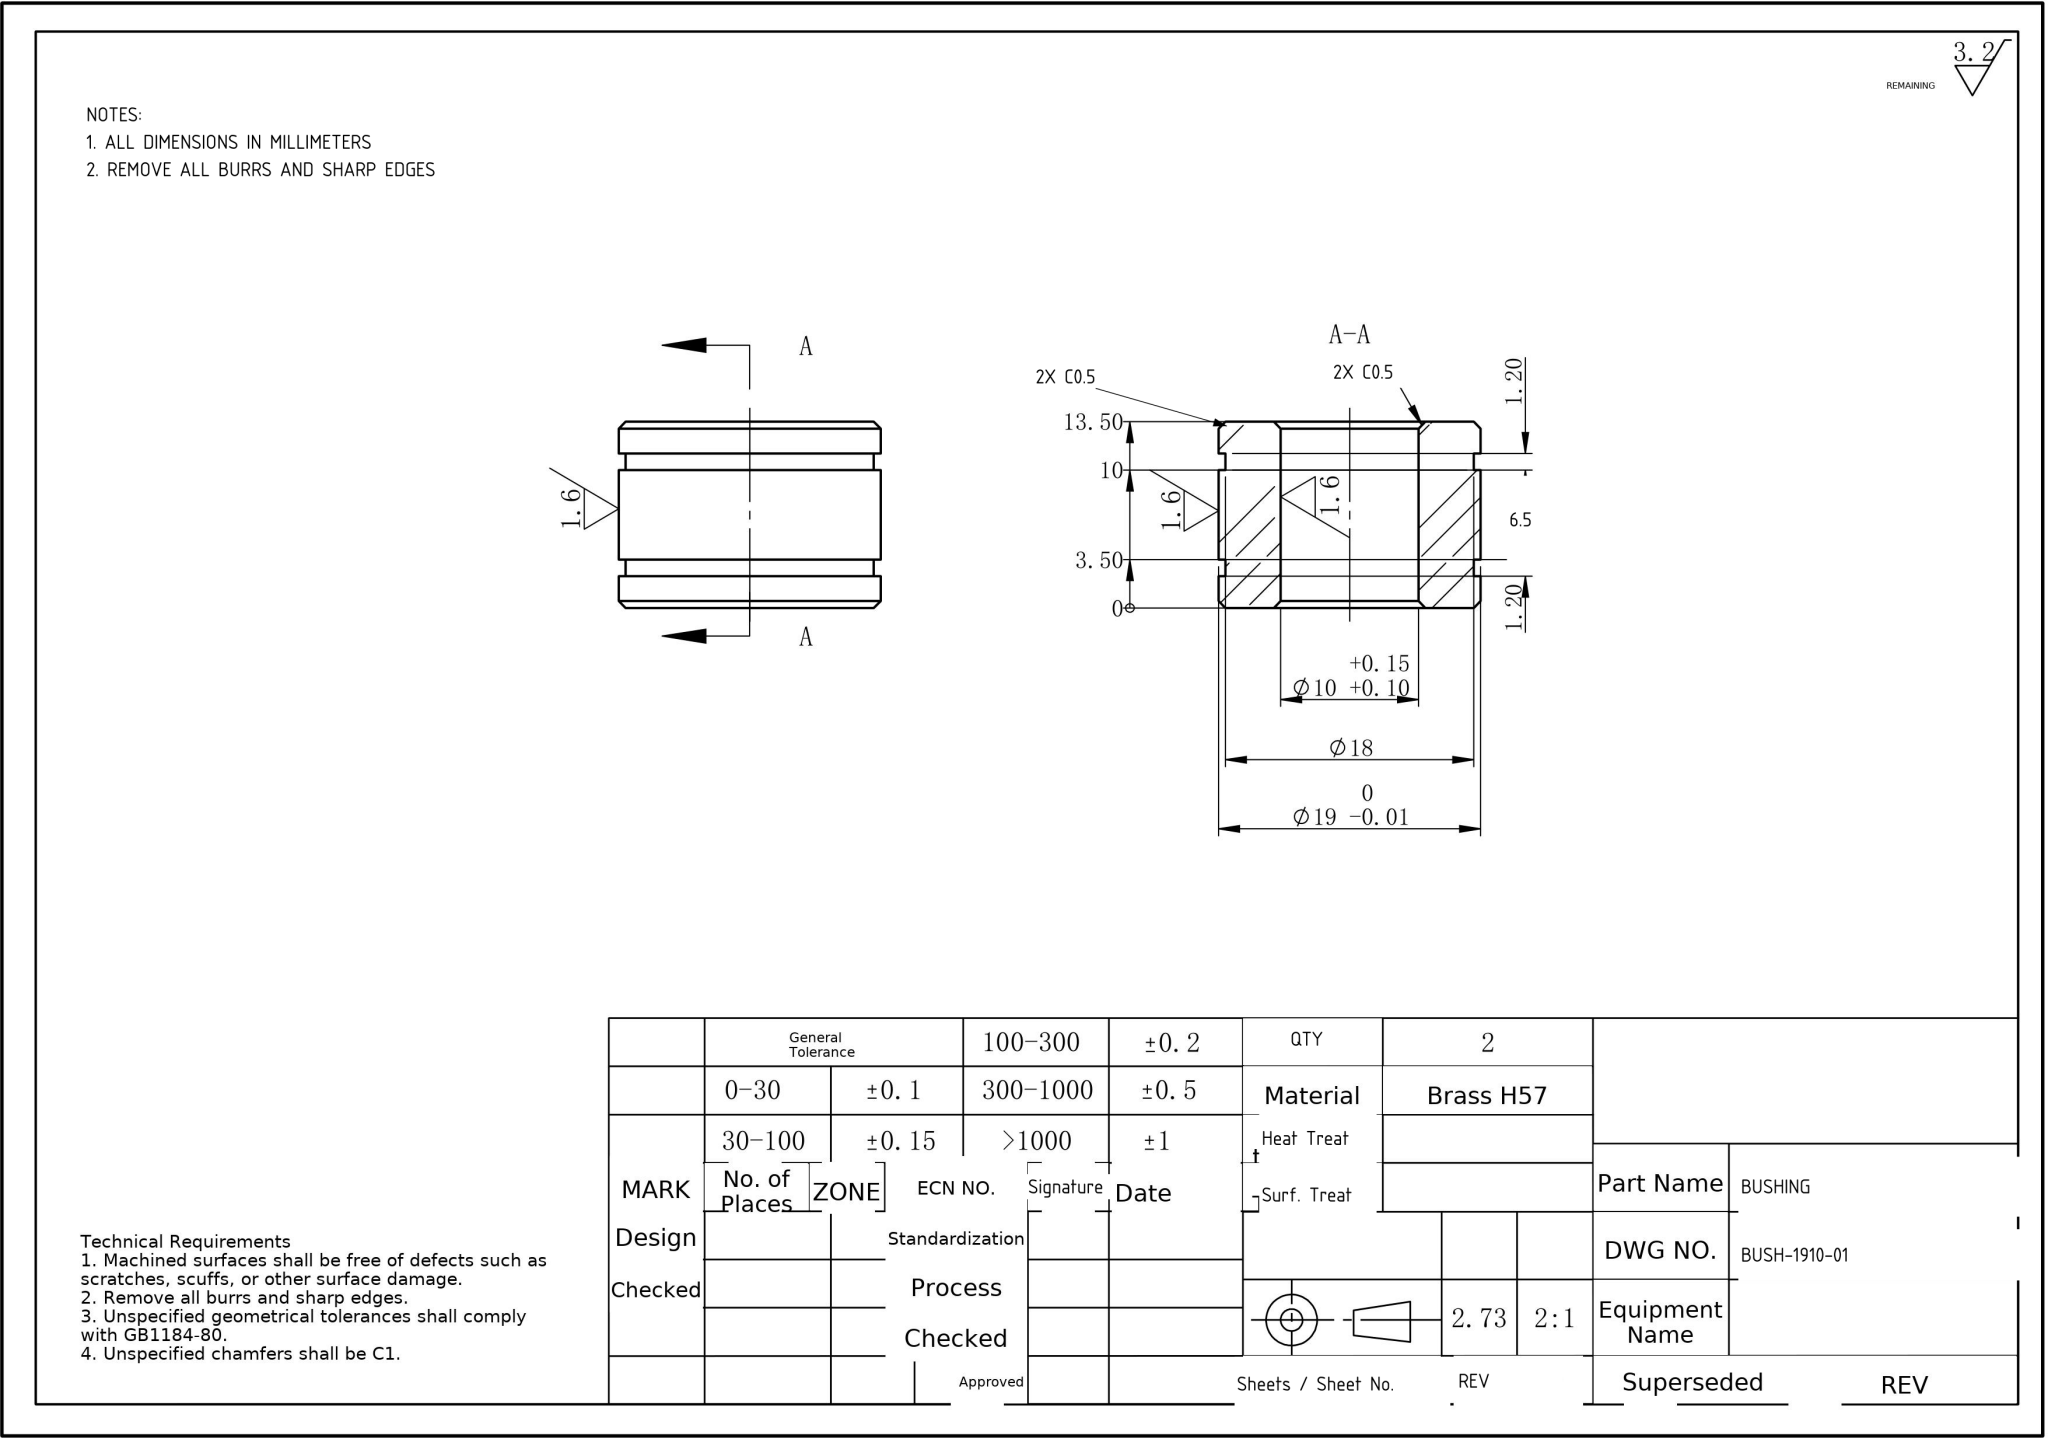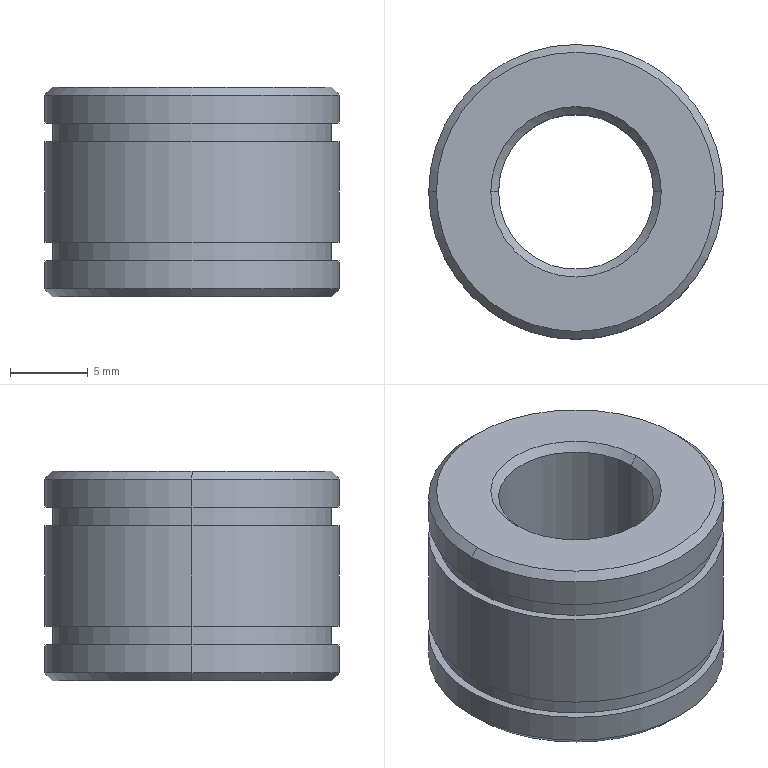Part | NX | mm | 1 solid | 26 faces | box 19 x 19 x 13.5 mm | volume 2675 mm3 | cylinder 12 | cone 8 | plane 6 | commonest cylinder face diameters 19 x6 18 x4 10 x2
STEP:
#1=COLOUR_RGB('',0.7922,0.8196,0.9333);
#2=FILL_AREA_STYLE_COLOUR('',#1);
#3=FILL_AREA_STYLE('',(#2));
#4=SURFACE_STYLE_FILL_AREA(#3);
#5=SURFACE_SIDE_STYLE('',(#4));
#6=SURFACE_STYLE_USAGE(.BOTH.,#5);
#7=PRESENTATION_STYLE_ASSIGNMENT((#6));
#8=CARTESIAN_POINT('',(-9.,0.,14.2));
#9=VERTEX_POINT('',#8);
#10=CARTESIAN_POINT('',(9.,0.,14.2));
#11=VERTEX_POINT('',#10);
#12=CARTESIAN_POINT('',(0.,0.,14.2));
#13=DIRECTION('',(0.,0.,-1.));
#14=DIRECTION('',(-1.,0.,0.));
#15=AXIS2_PLACEMENT_3D('',#12,#13,#14);
#16=CIRCLE('',#15,9.);
#17=EDGE_CURVE('',#9,#11,#16,.T.);
#18=ORIENTED_EDGE('',*,*,#17,.F.);
#19=CARTESIAN_POINT('',(-9.5,0.,14.7));
#20=VERTEX_POINT('',#19);
#21=CARTESIAN_POINT('',(-9.5,0.,14.7));
#22=DIRECTION('',(-0.7071,0.,0.7071));
#23=VECTOR('',#22,1000.);
#24=LINE('',#21,#23);
#25=EDGE_CURVE('',#9,#20,#24,.T.);
#26=ORIENTED_EDGE('',*,*,#25,.T.);
#27=CARTESIAN_POINT('',(9.5,0.,14.7));
#28=VERTEX_POINT('',#27);
#29=CARTESIAN_POINT('',(0.,0.,14.7));
#30=DIRECTION('',(0.,0.,1.));
#31=DIRECTION('',(-1.,0.,0.));
#32=AXIS2_PLACEMENT_3D('',#29,#30,#31);
#33=CIRCLE('',#32,9.5);
#34=EDGE_CURVE('',#28,#20,#33,.T.);
#35=ORIENTED_EDGE('',*,*,#34,.F.);
#36=CARTESIAN_POINT('',(9.5,0.,14.7));
#37=DIRECTION('',(0.7071,0.,0.7071));
#38=VECTOR('',#37,1000.);
#39=LINE('',#36,#38);
#40=EDGE_CURVE('',#11,#28,#39,.T.);
#41=ORIENTED_EDGE('',*,*,#40,.F.);
#42=EDGE_LOOP('',(#18,#26,#35,#41));
#43=FACE_OUTER_BOUND('',#42,.T.);
#44=CARTESIAN_POINT('',(0.,0.,14.7));
#45=DIRECTION('',(0.,0.,1.));
#46=DIRECTION('',(1.,0.,0.));
#47=AXIS2_PLACEMENT_3D('',#44,#45,#46);
#48=CONICAL_SURFACE('',#47,9.5,0.7854);
#49=ADVANCED_FACE('',(#43),#48,.T.);
#50=CARTESIAN_POINT('',(5.,0.,14.7));
#51=VERTEX_POINT('',#50);
#52=CARTESIAN_POINT('',(-5.,0.,14.7));
#53=VERTEX_POINT('',#52);
#54=CARTESIAN_POINT('',(0.,0.,14.7));
#55=DIRECTION('',(0.,0.,-1.));
#56=DIRECTION('',(-1.,0.,0.));
#57=AXIS2_PLACEMENT_3D('',#54,#55,#56);
#58=CIRCLE('',#57,5.);
#59=EDGE_CURVE('',#51,#53,#58,.T.);
#60=ORIENTED_EDGE('',*,*,#59,.F.);
#61=CARTESIAN_POINT('',(5.5,0.,14.2));
#62=VERTEX_POINT('',#61);
#63=CARTESIAN_POINT('',(5.5,0.,14.2));
#64=DIRECTION('',(0.7071,0.,-0.7071));
#65=VECTOR('',#64,1000.);
#66=LINE('',#63,#65);
#67=EDGE_CURVE('',#51,#62,#66,.T.);
#68=ORIENTED_EDGE('',*,*,#67,.T.);
#69=CARTESIAN_POINT('',(-5.5,0.,14.2));
#70=VERTEX_POINT('',#69);
#71=CARTESIAN_POINT('',(0.,0.,14.2));
#72=DIRECTION('',(0.,0.,1.));
#73=DIRECTION('',(-1.,0.,0.));
#74=AXIS2_PLACEMENT_3D('',#71,#72,#73);
#75=CIRCLE('',#74,5.5);
#76=EDGE_CURVE('',#70,#62,#75,.T.);
#77=ORIENTED_EDGE('',*,*,#76,.F.);
#78=CARTESIAN_POINT('',(-5.5,0.,14.2));
#79=DIRECTION('',(-0.7071,0.,-0.7071));
#80=VECTOR('',#79,1000.);
#81=LINE('',#78,#80);
#82=EDGE_CURVE('',#53,#70,#81,.T.);
#83=ORIENTED_EDGE('',*,*,#82,.F.);
#84=EDGE_LOOP('',(#60,#68,#77,#83));
#85=FACE_OUTER_BOUND('',#84,.T.);
#86=CARTESIAN_POINT('',(0.,0.,14.2));
#87=DIRECTION('',(0.,0.,-1.));
#88=DIRECTION('',(-1.,0.,0.));
#89=AXIS2_PLACEMENT_3D('',#86,#87,#88);
#90=CONICAL_SURFACE('',#89,5.5,0.7854);
#91=ADVANCED_FACE('',(#85),#90,.F.);
#92=CARTESIAN_POINT('',(9.,0.,27.7));
#93=VERTEX_POINT('',#92);
#94=CARTESIAN_POINT('',(-9.,0.,27.7));
#95=VERTEX_POINT('',#94);
#96=CARTESIAN_POINT('',(0.,0.,27.7));
#97=DIRECTION('',(0.,0.,1.));
#98=DIRECTION('',(1.,0.,0.));
#99=AXIS2_PLACEMENT_3D('',#96,#97,#98);
#100=CIRCLE('',#99,9.);
#101=EDGE_CURVE('',#93,#95,#100,.T.);
#102=ORIENTED_EDGE('',*,*,#101,.F.);
#103=CARTESIAN_POINT('',(9.5,0.,27.2));
#104=VERTEX_POINT('',#103);
#105=CARTESIAN_POINT('',(9.5,0.,27.2));
#106=DIRECTION('',(0.7071,0.,-0.7071));
#107=VECTOR('',#106,1000.);
#108=LINE('',#105,#107);
#109=EDGE_CURVE('',#93,#104,#108,.T.);
#110=ORIENTED_EDGE('',*,*,#109,.T.);
#111=CARTESIAN_POINT('',(-9.5,0.,27.2));
#112=VERTEX_POINT('',#111);
#113=CARTESIAN_POINT('',(0.,0.,27.2));
#114=DIRECTION('',(0.,0.,-1.));
#115=DIRECTION('',(1.,0.,0.));
#116=AXIS2_PLACEMENT_3D('',#113,#114,#115);
#117=CIRCLE('',#116,9.5);
#118=EDGE_CURVE('',#112,#104,#117,.T.);
#119=ORIENTED_EDGE('',*,*,#118,.F.);
#120=CARTESIAN_POINT('',(-9.5,0.,27.2));
#121=DIRECTION('',(-0.7071,0.,-0.7071));
#122=VECTOR('',#121,1000.);
#123=LINE('',#120,#122);
#124=EDGE_CURVE('',#95,#112,#123,.T.);
#125=ORIENTED_EDGE('',*,*,#124,.F.);
#126=EDGE_LOOP('',(#102,#110,#119,#125));
#127=FACE_OUTER_BOUND('',#126,.T.);
#128=CARTESIAN_POINT('',(0.,0.,27.2));
#129=DIRECTION('',(0.,0.,-1.));
#130=DIRECTION('',(-1.,0.,0.));
#131=AXIS2_PLACEMENT_3D('',#128,#129,#130);
#132=CONICAL_SURFACE('',#131,9.5,0.7854);
#133=ADVANCED_FACE('',(#127),#132,.T.);
#134=CARTESIAN_POINT('',(-5.,0.,27.2));
#135=VERTEX_POINT('',#134);
#136=CARTESIAN_POINT('',(5.,0.,27.2));
#137=VERTEX_POINT('',#136);
#138=CARTESIAN_POINT('',(0.,0.,27.2));
#139=DIRECTION('',(0.,0.,1.));
#140=DIRECTION('',(1.,0.,0.));
#141=AXIS2_PLACEMENT_3D('',#138,#139,#140);
#142=CIRCLE('',#141,5.);
#143=EDGE_CURVE('',#135,#137,#142,.T.);
#144=ORIENTED_EDGE('',*,*,#143,.F.);
#145=CARTESIAN_POINT('',(-5.5,0.,27.7));
#146=VERTEX_POINT('',#145);
#147=CARTESIAN_POINT('',(-5.5,0.,27.7));
#148=DIRECTION('',(-0.7071,0.,0.7071));
#149=VECTOR('',#148,1000.);
#150=LINE('',#147,#149);
#151=EDGE_CURVE('',#135,#146,#150,.T.);
#152=ORIENTED_EDGE('',*,*,#151,.T.);
#153=CARTESIAN_POINT('',(5.5,0.,27.7));
#154=VERTEX_POINT('',#153);
#155=CARTESIAN_POINT('',(0.,0.,27.7));
#156=DIRECTION('',(0.,0.,-1.));
#157=DIRECTION('',(1.,0.,0.));
#158=AXIS2_PLACEMENT_3D('',#155,#156,#157);
#159=CIRCLE('',#158,5.5);
#160=EDGE_CURVE('',#154,#146,#159,.T.);
#161=ORIENTED_EDGE('',*,*,#160,.F.);
#162=CARTESIAN_POINT('',(5.5,0.,27.7));
#163=DIRECTION('',(0.7071,0.,0.7071));
#164=VECTOR('',#163,1000.);
#165=LINE('',#162,#164);
#166=EDGE_CURVE('',#137,#154,#165,.T.);
#167=ORIENTED_EDGE('',*,*,#166,.F.);
#168=EDGE_LOOP('',(#144,#152,#161,#167));
#169=FACE_OUTER_BOUND('',#168,.T.);
#170=CARTESIAN_POINT('',(0.,0.,27.7));
#171=DIRECTION('',(0.,0.,1.));
#172=DIRECTION('',(1.,0.,0.));
#173=AXIS2_PLACEMENT_3D('',#170,#171,#172);
#174=CONICAL_SURFACE('',#173,5.5,0.7854);
#175=ADVANCED_FACE('',(#169),#174,.F.);
#176=CARTESIAN_POINT('',(9.,0.,16.5));
#177=VERTEX_POINT('',#176);
#178=CARTESIAN_POINT('',(-9.,0.,16.5));
#179=VERTEX_POINT('',#178);
#180=CARTESIAN_POINT('',(0.,0.,16.5));
#181=DIRECTION('',(0.,0.,1.));
#182=DIRECTION('',(1.,0.,0.));
#183=AXIS2_PLACEMENT_3D('',#180,#181,#182);
#184=CIRCLE('',#183,9.);
#185=EDGE_CURVE('',#177,#179,#184,.T.);
#186=ORIENTED_EDGE('',*,*,#185,.T.);
#187=CARTESIAN_POINT('',(-9.,0.,17.7));
#188=VERTEX_POINT('',#187);
#189=CARTESIAN_POINT('',(-9.,0.,12.9));
#190=DIRECTION('',(0.,0.,1.));
#191=VECTOR('',#190,1000.);
#192=LINE('',#189,#191);
#193=EDGE_CURVE('',#179,#188,#192,.T.);
#194=ORIENTED_EDGE('',*,*,#193,.T.);
#195=CARTESIAN_POINT('',(9.,0.,17.7));
#196=VERTEX_POINT('',#195);
#197=CARTESIAN_POINT('',(0.,0.,17.7));
#198=DIRECTION('',(0.,0.,1.));
#199=DIRECTION('',(1.,0.,0.));
#200=AXIS2_PLACEMENT_3D('',#197,#198,#199);
#201=CIRCLE('',#200,9.);
#202=EDGE_CURVE('',#196,#188,#201,.T.);
#203=ORIENTED_EDGE('',*,*,#202,.F.);
#204=CARTESIAN_POINT('',(9.,0.,12.9));
#205=DIRECTION('',(0.,0.,1.));
#206=VECTOR('',#205,1000.);
#207=LINE('',#204,#206);
#208=EDGE_CURVE('',#177,#196,#207,.T.);
#209=ORIENTED_EDGE('',*,*,#208,.F.);
#210=EDGE_LOOP('',(#186,#194,#203,#209));
#211=FACE_OUTER_BOUND('',#210,.T.);
#212=CARTESIAN_POINT('',(0.,0.,12.9));
#213=DIRECTION('',(0.,0.,1.));
#214=DIRECTION('',(1.,0.,0.));
#215=AXIS2_PLACEMENT_3D('',#212,#213,#214);
#216=CYLINDRICAL_SURFACE('',#215,9.);
#217=ADVANCED_FACE('',(#211),#216,.T.);
#218=CARTESIAN_POINT('',(-9.,0.,24.2));
#219=VERTEX_POINT('',#218);
#220=CARTESIAN_POINT('',(9.,0.,24.2));
#221=VERTEX_POINT('',#220);
#222=CARTESIAN_POINT('',(0.,0.,24.2));
#223=DIRECTION('',(0.,0.,-1.));
#224=DIRECTION('',(1.,0.,0.));
#225=AXIS2_PLACEMENT_3D('',#222,#223,#224);
#226=CIRCLE('',#225,9.);
#227=EDGE_CURVE('',#219,#221,#226,.T.);
#228=ORIENTED_EDGE('',*,*,#227,.F.);
#229=CARTESIAN_POINT('',(-9.,0.,25.4));
#230=VERTEX_POINT('',#229);
#231=CARTESIAN_POINT('',(-9.,0.,0.));
#232=DIRECTION('',(0.,0.,1.));
#233=VECTOR('',#232,1000.);
#234=LINE('',#231,#233);
#235=EDGE_CURVE('',#219,#230,#234,.T.);
#236=ORIENTED_EDGE('',*,*,#235,.T.);
#237=CARTESIAN_POINT('',(9.,0.,25.4));
#238=VERTEX_POINT('',#237);
#239=CARTESIAN_POINT('',(0.,0.,25.4));
#240=DIRECTION('',(0.,0.,-1.));
#241=DIRECTION('',(-1.,0.,0.));
#242=AXIS2_PLACEMENT_3D('',#239,#240,#241);
#243=CIRCLE('',#242,9.);
#244=EDGE_CURVE('',#230,#238,#243,.T.);
#245=ORIENTED_EDGE('',*,*,#244,.T.);
#246=CARTESIAN_POINT('',(9.,0.,0.));
#247=DIRECTION('',(0.,0.,1.));
#248=VECTOR('',#247,1000.);
#249=LINE('',#246,#248);
#250=EDGE_CURVE('',#221,#238,#249,.T.);
#251=ORIENTED_EDGE('',*,*,#250,.F.);
#252=EDGE_LOOP('',(#228,#236,#245,#251));
#253=FACE_OUTER_BOUND('',#252,.T.);
#254=CARTESIAN_POINT('',(0.,0.,0.));
#255=DIRECTION('',(0.,0.,1.));
#256=DIRECTION('',(1.,0.,0.));
#257=AXIS2_PLACEMENT_3D('',#254,#255,#256);
#258=CYLINDRICAL_SURFACE('',#257,9.);
#259=ADVANCED_FACE('',(#253),#258,.T.);
#260=CARTESIAN_POINT('',(9.5,0.,17.7));
#261=VERTEX_POINT('',#260);
#262=CARTESIAN_POINT('',(-9.5,0.,17.7));
#263=VERTEX_POINT('',#262);
#264=CARTESIAN_POINT('',(0.,0.,17.7));
#265=DIRECTION('',(0.,0.,1.));
#266=DIRECTION('',(1.,0.,0.));
#267=AXIS2_PLACEMENT_3D('',#264,#265,#266);
#268=CIRCLE('',#267,9.5);
#269=EDGE_CURVE('',#261,#263,#268,.T.);
#270=ORIENTED_EDGE('',*,*,#269,.T.);
#271=CARTESIAN_POINT('',(-9.5,0.,24.2));
#272=VERTEX_POINT('',#271);
#273=CARTESIAN_POINT('',(-9.5,0.,0.));
#274=DIRECTION('',(0.,0.,1.));
#275=VECTOR('',#274,1000.);
#276=LINE('',#273,#275);
#277=EDGE_CURVE('',#263,#272,#276,.T.);
#278=ORIENTED_EDGE('',*,*,#277,.T.);
#279=CARTESIAN_POINT('',(9.5,0.,24.2));
#280=VERTEX_POINT('',#279);
#281=CARTESIAN_POINT('',(0.,0.,24.2));
#282=DIRECTION('',(0.,0.,-1.));
#283=DIRECTION('',(1.,0.,0.));
#284=AXIS2_PLACEMENT_3D('',#281,#282,#283);
#285=CIRCLE('',#284,9.5);
#286=EDGE_CURVE('',#272,#280,#285,.T.);
#287=ORIENTED_EDGE('',*,*,#286,.T.);
#288=CARTESIAN_POINT('',(9.5,0.,0.));
#289=DIRECTION('',(0.,0.,1.));
#290=VECTOR('',#289,1000.);
#291=LINE('',#288,#290);
#292=EDGE_CURVE('',#261,#280,#291,.T.);
#293=ORIENTED_EDGE('',*,*,#292,.F.);
#294=EDGE_LOOP('',(#270,#278,#287,#293));
#295=FACE_OUTER_BOUND('',#294,.T.);
#296=CARTESIAN_POINT('',(0.,0.,0.));
#297=DIRECTION('',(0.,0.,1.));
#298=DIRECTION('',(1.,0.,0.));
#299=AXIS2_PLACEMENT_3D('',#296,#297,#298);
#300=CYLINDRICAL_SURFACE('',#299,9.5);
#301=ADVANCED_FACE('',(#295),#300,.T.);
#302=ORIENTED_EDGE('',*,*,#34,.T.);
#303=CARTESIAN_POINT('',(-9.5,0.,16.5));
#304=VERTEX_POINT('',#303);
#305=CARTESIAN_POINT('',(-9.5,0.,12.9));
#306=DIRECTION('',(0.,0.,1.));
#307=VECTOR('',#306,1000.);
#308=LINE('',#305,#307);
#309=EDGE_CURVE('',#20,#304,#308,.T.);
#310=ORIENTED_EDGE('',*,*,#309,.T.);
#311=CARTESIAN_POINT('',(9.5,0.,16.5));
#312=VERTEX_POINT('',#311);
#313=CARTESIAN_POINT('',(0.,0.,16.5));
#314=DIRECTION('',(0.,0.,1.));
#315=DIRECTION('',(1.,0.,0.));
#316=AXIS2_PLACEMENT_3D('',#313,#314,#315);
#317=CIRCLE('',#316,9.5);
#318=EDGE_CURVE('',#312,#304,#317,.T.);
#319=ORIENTED_EDGE('',*,*,#318,.F.);
#320=CARTESIAN_POINT('',(9.5,0.,12.9));
#321=DIRECTION('',(0.,0.,1.));
#322=VECTOR('',#321,1000.);
#323=LINE('',#320,#322);
#324=EDGE_CURVE('',#28,#312,#323,.T.);
#325=ORIENTED_EDGE('',*,*,#324,.F.);
#326=EDGE_LOOP('',(#302,#310,#319,#325));
#327=FACE_OUTER_BOUND('',#326,.T.);
#328=CARTESIAN_POINT('',(0.,0.,12.9));
#329=DIRECTION('',(0.,0.,1.));
#330=DIRECTION('',(1.,0.,0.));
#331=AXIS2_PLACEMENT_3D('',#328,#329,#330);
#332=CYLINDRICAL_SURFACE('',#331,9.5);
#333=ADVANCED_FACE('',(#327),#332,.T.);
#334=CARTESIAN_POINT('',(-9.5,0.,25.4));
#335=VERTEX_POINT('',#334);
#336=CARTESIAN_POINT('',(9.5,0.,25.4));
#337=VERTEX_POINT('',#336);
#338=CARTESIAN_POINT('',(0.,0.,25.4));
#339=DIRECTION('',(0.,0.,-1.));
#340=DIRECTION('',(-1.,0.,0.));
#341=AXIS2_PLACEMENT_3D('',#338,#339,#340);
#342=CIRCLE('',#341,9.5);
#343=EDGE_CURVE('',#335,#337,#342,.T.);
#344=ORIENTED_EDGE('',*,*,#343,.F.);
#345=CARTESIAN_POINT('',(-9.5,0.,0.));
#346=DIRECTION('',(0.,0.,1.));
#347=VECTOR('',#346,1000.);
#348=LINE('',#345,#347);
#349=EDGE_CURVE('',#335,#112,#348,.T.);
#350=ORIENTED_EDGE('',*,*,#349,.T.);
#351=ORIENTED_EDGE('',*,*,#118,.T.);
#352=CARTESIAN_POINT('',(9.5,0.,0.));
#353=DIRECTION('',(0.,0.,1.));
#354=VECTOR('',#353,1000.);
#355=LINE('',#352,#354);
#356=EDGE_CURVE('',#337,#104,#355,.T.);
#357=ORIENTED_EDGE('',*,*,#356,.F.);
#358=EDGE_LOOP('',(#344,#350,#351,#357));
#359=FACE_OUTER_BOUND('',#358,.T.);
#360=CARTESIAN_POINT('',(0.,0.,0.));
#361=DIRECTION('',(0.,0.,1.));
#362=DIRECTION('',(1.,0.,0.));
#363=AXIS2_PLACEMENT_3D('',#360,#361,#362);
#364=CYLINDRICAL_SURFACE('',#363,9.5);
#365=ADVANCED_FACE('',(#359),#364,.T.);
#366=ORIENTED_EDGE('',*,*,#59,.T.);
#367=CARTESIAN_POINT('',(-5.,0.,0.));
#368=DIRECTION('',(0.,0.,1.));
#369=VECTOR('',#368,1000.);
#370=LINE('',#367,#369);
#371=EDGE_CURVE('',#53,#135,#370,.T.);
#372=ORIENTED_EDGE('',*,*,#371,.T.);
#373=ORIENTED_EDGE('',*,*,#143,.T.);
#374=CARTESIAN_POINT('',(5.,0.,0.));
#375=DIRECTION('',(0.,0.,1.));
#376=VECTOR('',#375,1000.);
#377=LINE('',#374,#376);
#378=EDGE_CURVE('',#51,#137,#377,.T.);
#379=ORIENTED_EDGE('',*,*,#378,.F.);
#380=EDGE_LOOP('',(#366,#372,#373,#379));
#381=FACE_OUTER_BOUND('',#380,.T.);
#382=CARTESIAN_POINT('',(0.,0.,0.));
#383=DIRECTION('',(0.,0.,1.));
#384=DIRECTION('',(1.,0.,0.));
#385=AXIS2_PLACEMENT_3D('',#382,#383,#384);
#386=CYLINDRICAL_SURFACE('',#385,5.);
#387=ADVANCED_FACE('',(#381),#386,.F.);
#388=ORIENTED_EDGE('',*,*,#371,.F.);
#389=CARTESIAN_POINT('',(0.,0.,14.7));
#390=DIRECTION('',(0.,0.,-1.));
#391=DIRECTION('',(-1.,0.,0.));
#392=AXIS2_PLACEMENT_3D('',#389,#390,#391);
#393=CIRCLE('',#392,5.);
#394=EDGE_CURVE('',#53,#51,#393,.T.);
#395=ORIENTED_EDGE('',*,*,#394,.T.);
#396=ORIENTED_EDGE('',*,*,#378,.T.);
#397=CARTESIAN_POINT('',(0.,0.,27.2));
#398=DIRECTION('',(0.,0.,1.));
#399=DIRECTION('',(1.,0.,0.));
#400=AXIS2_PLACEMENT_3D('',#397,#398,#399);
#401=CIRCLE('',#400,5.);
#402=EDGE_CURVE('',#137,#135,#401,.T.);
#403=ORIENTED_EDGE('',*,*,#402,.T.);
#404=EDGE_LOOP('',(#388,#395,#396,#403));
#405=FACE_OUTER_BOUND('',#404,.T.);
#406=CARTESIAN_POINT('',(0.,0.,0.));
#407=DIRECTION('',(0.,0.,1.));
#408=DIRECTION('',(1.,0.,0.));
#409=AXIS2_PLACEMENT_3D('',#406,#407,#408);
#410=CYLINDRICAL_SURFACE('',#409,5.);
#411=ADVANCED_FACE('',(#405),#410,.F.);
#412=ORIENTED_EDGE('',*,*,#349,.F.);
#413=CARTESIAN_POINT('',(0.,0.,25.4));
#414=DIRECTION('',(0.,0.,-1.));
#415=DIRECTION('',(-1.,0.,0.));
#416=AXIS2_PLACEMENT_3D('',#413,#414,#415);
#417=CIRCLE('',#416,9.5);
#418=EDGE_CURVE('',#337,#335,#417,.T.);
#419=ORIENTED_EDGE('',*,*,#418,.F.);
#420=ORIENTED_EDGE('',*,*,#356,.T.);
#421=CARTESIAN_POINT('',(0.,0.,27.2));
#422=DIRECTION('',(0.,0.,-1.));
#423=DIRECTION('',(1.,0.,0.));
#424=AXIS2_PLACEMENT_3D('',#421,#422,#423);
#425=CIRCLE('',#424,9.5);
#426=EDGE_CURVE('',#104,#112,#425,.T.);
#427=ORIENTED_EDGE('',*,*,#426,.T.);
#428=EDGE_LOOP('',(#412,#419,#420,#427));
#429=FACE_OUTER_BOUND('',#428,.T.);
#430=CARTESIAN_POINT('',(0.,0.,0.));
#431=DIRECTION('',(0.,0.,1.));
#432=DIRECTION('',(1.,0.,0.));
#433=AXIS2_PLACEMENT_3D('',#430,#431,#432);
#434=CYLINDRICAL_SURFACE('',#433,9.5);
#435=ADVANCED_FACE('',(#429),#434,.T.);
#436=ORIENTED_EDGE('',*,*,#309,.F.);
#437=CARTESIAN_POINT('',(0.,0.,14.7));
#438=DIRECTION('',(0.,0.,1.));
#439=DIRECTION('',(-1.,0.,0.));
#440=AXIS2_PLACEMENT_3D('',#437,#438,#439);
#441=CIRCLE('',#440,9.5);
#442=EDGE_CURVE('',#20,#28,#441,.T.);
#443=ORIENTED_EDGE('',*,*,#442,.T.);
#444=ORIENTED_EDGE('',*,*,#324,.T.);
#445=CARTESIAN_POINT('',(0.,0.,16.5));
#446=DIRECTION('',(0.,0.,1.));
#447=DIRECTION('',(1.,0.,0.));
#448=AXIS2_PLACEMENT_3D('',#445,#446,#447);
#449=CIRCLE('',#448,9.5);
#450=EDGE_CURVE('',#304,#312,#449,.T.);
#451=ORIENTED_EDGE('',*,*,#450,.F.);
#452=EDGE_LOOP('',(#436,#443,#444,#451));
#453=FACE_OUTER_BOUND('',#452,.T.);
#454=CARTESIAN_POINT('',(0.,0.,12.9));
#455=DIRECTION('',(0.,0.,1.));
#456=DIRECTION('',(1.,0.,0.));
#457=AXIS2_PLACEMENT_3D('',#454,#455,#456);
#458=CYLINDRICAL_SURFACE('',#457,9.5);
#459=ADVANCED_FACE('',(#453),#458,.T.);
#460=ORIENTED_EDGE('',*,*,#277,.F.);
#461=CARTESIAN_POINT('',(0.,0.,17.7));
#462=DIRECTION('',(0.,0.,1.));
#463=DIRECTION('',(1.,0.,0.));
#464=AXIS2_PLACEMENT_3D('',#461,#462,#463);
#465=CIRCLE('',#464,9.5);
#466=EDGE_CURVE('',#263,#261,#465,.T.);
#467=ORIENTED_EDGE('',*,*,#466,.T.);
#468=ORIENTED_EDGE('',*,*,#292,.T.);
#469=CARTESIAN_POINT('',(0.,0.,24.2));
#470=DIRECTION('',(0.,0.,-1.));
#471=DIRECTION('',(1.,0.,0.));
#472=AXIS2_PLACEMENT_3D('',#469,#470,#471);
#473=CIRCLE('',#472,9.5);
#474=EDGE_CURVE('',#280,#272,#473,.T.);
#475=ORIENTED_EDGE('',*,*,#474,.T.);
#476=EDGE_LOOP('',(#460,#467,#468,#475));
#477=FACE_OUTER_BOUND('',#476,.T.);
#478=CARTESIAN_POINT('',(0.,0.,0.));
#479=DIRECTION('',(0.,0.,1.));
#480=DIRECTION('',(1.,0.,0.));
#481=AXIS2_PLACEMENT_3D('',#478,#479,#480);
#482=CYLINDRICAL_SURFACE('',#481,9.5);
#483=ADVANCED_FACE('',(#477),#482,.T.);
#484=ORIENTED_EDGE('',*,*,#474,.F.);
#485=ORIENTED_EDGE('',*,*,#286,.F.);
#486=EDGE_LOOP('',(#484,#485));
#487=FACE_OUTER_BOUND('',#486,.T.);
#488=CARTESIAN_POINT('',(0.,0.,24.2));
#489=DIRECTION('',(0.,0.,-1.));
#490=DIRECTION('',(1.,0.,0.));
#491=AXIS2_PLACEMENT_3D('',#488,#489,#490);
#492=CIRCLE('',#491,9.);
#493=EDGE_CURVE('',#221,#219,#492,.T.);
#494=ORIENTED_EDGE('',*,*,#493,.T.);
#495=ORIENTED_EDGE('',*,*,#227,.T.);
#496=EDGE_LOOP('',(#494,#495));
#497=FACE_BOUND('',#496,.T.);
#498=CARTESIAN_POINT('',(0.,9.5,24.2));
#499=DIRECTION('',(0.,0.,1.));
#500=DIRECTION('',(1.,0.,0.));
#501=AXIS2_PLACEMENT_3D('',#498,#499,#500);
#502=PLANE('',#501);
#503=ADVANCED_FACE('',(#487,#497),#502,.T.);
#504=ORIENTED_EDGE('',*,*,#235,.F.);
#505=ORIENTED_EDGE('',*,*,#493,.F.);
#506=ORIENTED_EDGE('',*,*,#250,.T.);
#507=CARTESIAN_POINT('',(0.,0.,25.4));
#508=DIRECTION('',(0.,0.,-1.));
#509=DIRECTION('',(-1.,0.,0.));
#510=AXIS2_PLACEMENT_3D('',#507,#508,#509);
#511=CIRCLE('',#510,9.);
#512=EDGE_CURVE('',#238,#230,#511,.T.);
#513=ORIENTED_EDGE('',*,*,#512,.T.);
#514=EDGE_LOOP('',(#504,#505,#506,#513));
#515=FACE_OUTER_BOUND('',#514,.T.);
#516=CARTESIAN_POINT('',(0.,0.,0.));
#517=DIRECTION('',(0.,0.,1.));
#518=DIRECTION('',(1.,0.,0.));
#519=AXIS2_PLACEMENT_3D('',#516,#517,#518);
#520=CYLINDRICAL_SURFACE('',#519,9.);
#521=ADVANCED_FACE('',(#515),#520,.T.);
#522=ORIENTED_EDGE('',*,*,#512,.F.);
#523=ORIENTED_EDGE('',*,*,#244,.F.);
#524=EDGE_LOOP('',(#522,#523));
#525=FACE_BOUND('',#524,.T.);
#526=ORIENTED_EDGE('',*,*,#418,.T.);
#527=ORIENTED_EDGE('',*,*,#343,.T.);
#528=EDGE_LOOP('',(#526,#527));
#529=FACE_OUTER_BOUND('',#528,.T.);
#530=CARTESIAN_POINT('',(0.,9.,25.4));
#531=DIRECTION('',(0.,0.,-1.));
#532=DIRECTION('',(-1.,0.,0.));
#533=AXIS2_PLACEMENT_3D('',#530,#531,#532);
#534=PLANE('',#533);
#535=ADVANCED_FACE('',(#525,#529),#534,.T.);
#536=ORIENTED_EDGE('',*,*,#318,.T.);
#537=ORIENTED_EDGE('',*,*,#450,.T.);
#538=EDGE_LOOP('',(#536,#537));
#539=FACE_OUTER_BOUND('',#538,.T.);
#540=ORIENTED_EDGE('',*,*,#185,.F.);
#541=CARTESIAN_POINT('',(0.,0.,16.5));
#542=DIRECTION('',(0.,0.,1.));
#543=DIRECTION('',(1.,0.,0.));
#544=AXIS2_PLACEMENT_3D('',#541,#542,#543);
#545=CIRCLE('',#544,9.);
#546=EDGE_CURVE('',#179,#177,#545,.T.);
#547=ORIENTED_EDGE('',*,*,#546,.F.);
#548=EDGE_LOOP('',(#540,#547));
#549=FACE_BOUND('',#548,.T.);
#550=CARTESIAN_POINT('',(0.,9.5,16.5));
#551=DIRECTION('',(0.,0.,1.));
#552=DIRECTION('',(1.,0.,0.));
#553=AXIS2_PLACEMENT_3D('',#550,#551,#552);
#554=PLANE('',#553);
#555=ADVANCED_FACE('',(#539,#549),#554,.T.);
#556=ORIENTED_EDGE('',*,*,#193,.F.);
#557=ORIENTED_EDGE('',*,*,#546,.T.);
#558=ORIENTED_EDGE('',*,*,#208,.T.);
#559=CARTESIAN_POINT('',(0.,0.,17.7));
#560=DIRECTION('',(0.,0.,1.));
#561=DIRECTION('',(1.,0.,0.));
#562=AXIS2_PLACEMENT_3D('',#559,#560,#561);
#563=CIRCLE('',#562,9.);
#564=EDGE_CURVE('',#188,#196,#563,.T.);
#565=ORIENTED_EDGE('',*,*,#564,.F.);
#566=EDGE_LOOP('',(#556,#557,#558,#565));
#567=FACE_OUTER_BOUND('',#566,.T.);
#568=CARTESIAN_POINT('',(0.,0.,12.9));
#569=DIRECTION('',(0.,0.,1.));
#570=DIRECTION('',(1.,0.,0.));
#571=AXIS2_PLACEMENT_3D('',#568,#569,#570);
#572=CYLINDRICAL_SURFACE('',#571,9.);
#573=ADVANCED_FACE('',(#567),#572,.T.);
#574=ORIENTED_EDGE('',*,*,#202,.T.);
#575=ORIENTED_EDGE('',*,*,#564,.T.);
#576=EDGE_LOOP('',(#574,#575));
#577=FACE_BOUND('',#576,.T.);
#578=ORIENTED_EDGE('',*,*,#269,.F.);
#579=ORIENTED_EDGE('',*,*,#466,.F.);
#580=EDGE_LOOP('',(#578,#579));
#581=FACE_OUTER_BOUND('',#580,.T.);
#582=CARTESIAN_POINT('',(0.,9.,17.7));
#583=DIRECTION('',(0.,0.,-1.));
#584=DIRECTION('',(-1.,0.,0.));
#585=AXIS2_PLACEMENT_3D('',#582,#583,#584);
#586=PLANE('',#585);
#587=ADVANCED_FACE('',(#577,#581),#586,.T.);
#588=ORIENTED_EDGE('',*,*,#76,.T.);
#589=CARTESIAN_POINT('',(0.,0.,14.2));
#590=DIRECTION('',(0.,0.,1.));
#591=DIRECTION('',(-1.,0.,0.));
#592=AXIS2_PLACEMENT_3D('',#589,#590,#591);
#593=CIRCLE('',#592,5.5);
#594=EDGE_CURVE('',#62,#70,#593,.T.);
#595=ORIENTED_EDGE('',*,*,#594,.T.);
#596=EDGE_LOOP('',(#588,#595));
#597=FACE_BOUND('',#596,.T.);
#598=CARTESIAN_POINT('',(0.,0.,14.2));
#599=DIRECTION('',(0.,0.,-1.));
#600=DIRECTION('',(-1.,0.,0.));
#601=AXIS2_PLACEMENT_3D('',#598,#599,#600);
#602=CIRCLE('',#601,9.);
#603=EDGE_CURVE('',#11,#9,#602,.T.);
#604=ORIENTED_EDGE('',*,*,#603,.T.);
#605=ORIENTED_EDGE('',*,*,#17,.T.);
#606=EDGE_LOOP('',(#604,#605));
#607=FACE_OUTER_BOUND('',#606,.T.);
#608=CARTESIAN_POINT('',(0.,0.,14.2));
#609=DIRECTION('',(0.,0.,-1.));
#610=DIRECTION('',(-1.,0.,0.));
#611=AXIS2_PLACEMENT_3D('',#608,#609,#610);
#612=PLANE('',#611);
#613=ADVANCED_FACE('',(#597,#607),#612,.T.);
#614=ORIENTED_EDGE('',*,*,#160,.T.);
#615=CARTESIAN_POINT('',(0.,0.,27.7));
#616=DIRECTION('',(0.,0.,-1.));
#617=DIRECTION('',(1.,0.,0.));
#618=AXIS2_PLACEMENT_3D('',#615,#616,#617);
#619=CIRCLE('',#618,5.5);
#620=EDGE_CURVE('',#146,#154,#619,.T.);
#621=ORIENTED_EDGE('',*,*,#620,.T.);
#622=EDGE_LOOP('',(#614,#621));
#623=FACE_BOUND('',#622,.T.);
#624=CARTESIAN_POINT('',(0.,0.,27.7));
#625=DIRECTION('',(0.,0.,1.));
#626=DIRECTION('',(1.,0.,0.));
#627=AXIS2_PLACEMENT_3D('',#624,#625,#626);
#628=CIRCLE('',#627,9.);
#629=EDGE_CURVE('',#95,#93,#628,.T.);
#630=ORIENTED_EDGE('',*,*,#629,.T.);
#631=ORIENTED_EDGE('',*,*,#101,.T.);
#632=EDGE_LOOP('',(#630,#631));
#633=FACE_OUTER_BOUND('',#632,.T.);
#634=CARTESIAN_POINT('',(0.,0.,27.7));
#635=DIRECTION('',(0.,0.,1.));
#636=DIRECTION('',(1.,0.,0.));
#637=AXIS2_PLACEMENT_3D('',#634,#635,#636);
#638=PLANE('',#637);
#639=ADVANCED_FACE('',(#623,#633),#638,.T.);
#640=ORIENTED_EDGE('',*,*,#151,.F.);
#641=ORIENTED_EDGE('',*,*,#402,.F.);
#642=ORIENTED_EDGE('',*,*,#166,.T.);
#643=ORIENTED_EDGE('',*,*,#620,.F.);
#644=EDGE_LOOP('',(#640,#641,#642,#643));
#645=FACE_OUTER_BOUND('',#644,.T.);
#646=CARTESIAN_POINT('',(0.,0.,27.7));
#647=DIRECTION('',(0.,0.,1.));
#648=DIRECTION('',(1.,0.,0.));
#649=AXIS2_PLACEMENT_3D('',#646,#647,#648);
#650=CONICAL_SURFACE('',#649,5.5,0.7854);
#651=ADVANCED_FACE('',(#645),#650,.F.);
#652=ORIENTED_EDGE('',*,*,#109,.F.);
#653=ORIENTED_EDGE('',*,*,#629,.F.);
#654=ORIENTED_EDGE('',*,*,#124,.T.);
#655=ORIENTED_EDGE('',*,*,#426,.F.);
#656=EDGE_LOOP('',(#652,#653,#654,#655));
#657=FACE_OUTER_BOUND('',#656,.T.);
#658=CARTESIAN_POINT('',(0.,0.,27.2));
#659=DIRECTION('',(0.,0.,-1.));
#660=DIRECTION('',(-1.,0.,0.));
#661=AXIS2_PLACEMENT_3D('',#658,#659,#660);
#662=CONICAL_SURFACE('',#661,9.5,0.7854);
#663=ADVANCED_FACE('',(#657),#662,.T.);
#664=ORIENTED_EDGE('',*,*,#67,.F.);
#665=ORIENTED_EDGE('',*,*,#394,.F.);
#666=ORIENTED_EDGE('',*,*,#82,.T.);
#667=ORIENTED_EDGE('',*,*,#594,.F.);
#668=EDGE_LOOP('',(#664,#665,#666,#667));
#669=FACE_OUTER_BOUND('',#668,.T.);
#670=CARTESIAN_POINT('',(0.,0.,14.2));
#671=DIRECTION('',(0.,0.,-1.));
#672=DIRECTION('',(-1.,0.,0.));
#673=AXIS2_PLACEMENT_3D('',#670,#671,#672);
#674=CONICAL_SURFACE('',#673,5.5,0.7854);
#675=ADVANCED_FACE('',(#669),#674,.F.);
#676=ORIENTED_EDGE('',*,*,#25,.F.);
#677=ORIENTED_EDGE('',*,*,#603,.F.);
#678=ORIENTED_EDGE('',*,*,#40,.T.);
#679=ORIENTED_EDGE('',*,*,#442,.F.);
#680=EDGE_LOOP('',(#676,#677,#678,#679));
#681=FACE_OUTER_BOUND('',#680,.T.);
#682=CARTESIAN_POINT('',(0.,0.,14.7));
#683=DIRECTION('',(0.,0.,1.));
#684=DIRECTION('',(1.,0.,0.));
#685=AXIS2_PLACEMENT_3D('',#682,#683,#684);
#686=CONICAL_SURFACE('',#685,9.5,0.7854);
#687=ADVANCED_FACE('',(#681),#686,.T.);
#688=CLOSED_SHELL('',(#49,#91,#133,#175,#217,#259,#301,#333,#365,#387,#411,#435,#459,#483,#503,#521,#535,#555,#573,#587,#613,#639,#651,#663,#675,#687));
#689=MANIFOLD_SOLID_BREP('',#688);
#690=STYLED_ITEM('',(#7),#689);
#691=(LENGTH_UNIT()NAMED_UNIT(*)SI_UNIT(.MILLI.,.METRE.));
#692=UNCERTAINTY_MEASURE_WITH_UNIT(LENGTH_MEASURE(0.00001),#691,'','');
#693=(NAMED_UNIT(*)PLANE_ANGLE_UNIT()SI_UNIT($,.RADIAN.));
#694=(NAMED_UNIT(*)SI_UNIT($,.STERADIAN.)SOLID_ANGLE_UNIT());
#695=(GEOMETRIC_REPRESENTATION_CONTEXT(3)GLOBAL_UNCERTAINTY_ASSIGNED_CONTEXT((#692))GLOBAL_UNIT_ASSIGNED_CONTEXT((#691,#693,#694))REPRESENTATION_CONTEXT('',''));
#696=MECHANICAL_DESIGN_GEOMETRIC_PRESENTATION_REPRESENTATION('',(#690),#695);
#697=PRESENTATION_LAYER_ASSIGNMENT('','',(#690));
#698=CARTESIAN_POINT('',(0.,0.,0.));
#699=DIRECTION('',(0.,0.,1.));
#700=DIRECTION('',(1.,0.,0.));
#701=AXIS2_PLACEMENT_3D('',#698,#699,#700);
#702=(LENGTH_UNIT()NAMED_UNIT(*)SI_UNIT(.MILLI.,.METRE.));
#703=UNCERTAINTY_MEASURE_WITH_UNIT(LENGTH_MEASURE(0.00001),#702,'','');
#704=(NAMED_UNIT(*)PLANE_ANGLE_UNIT()SI_UNIT($,.RADIAN.));
#705=(NAMED_UNIT(*)SI_UNIT($,.STERADIAN.)SOLID_ANGLE_UNIT());
#706=(GEOMETRIC_REPRESENTATION_CONTEXT(3)GLOBAL_UNCERTAINTY_ASSIGNED_CONTEXT((#703))GLOBAL_UNIT_ASSIGNED_CONTEXT((#702,#704,#705))REPRESENTATION_CONTEXT('',''));
#707=ADVANCED_BREP_SHAPE_REPRESENTATION('',(#689,#701),#706);